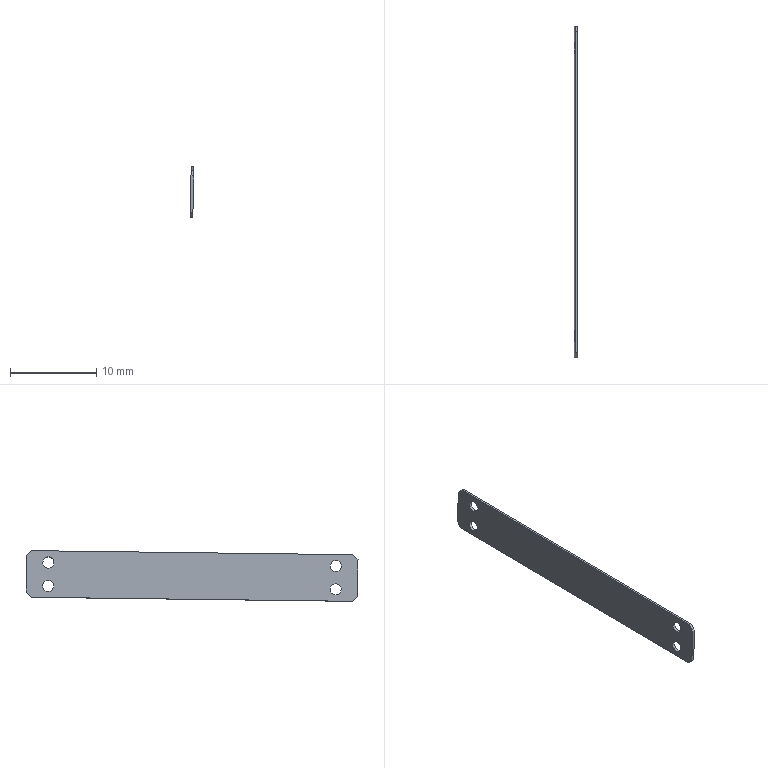Component | SolidWorks | 00-VacuumSuctionCupAssembly-1_11-RetainingPlate-2 | 1 solid | 18 faces | box 0.4 x 38.45 x 5.87 mm | volume 60 mm3 | plane 10 | cylinder 8 | commonest cylinder face diameters 1.29 x8
build123d program:
from build123d import *

# Parameters (mm, degrees)
SKETCH1_R           = 2.15
BOSS_EXTRUDE1_DEPTH = 1
SCALE1_SCALE        = 0.3


with BuildPart() as part:
    # Sketch1 → Boss-Extrude1 (new body)
    with BuildSketch(Plane(origin=(1, 0, 0), x_dir=(0, 0, -1), z_dir=(1, 0, 0))):
        Polygon((-64, 7), (-64, -7), (-62, -9), (62, -9), (64, -7), (64, 7), (62, 9), (-62, 9), align=None)
        with Locations(Location((-55.5, 4.5, 0), (0, 0, 180))):
            Circle(SKETCH1_R, mode=Mode.SUBTRACT)
        with Locations(Location((-55.5, -4.5, 0), (0, 0, 180))):
            Circle(SKETCH1_R, mode=Mode.SUBTRACT)
        with Locations(Location((55.5, 4.5, 0), (0, 0, 180))):
            Circle(SKETCH1_R, mode=Mode.SUBTRACT)
        with Locations(Location((55.5, -4.5, 0), (0, 0, 180))):
            Circle(SKETCH1_R, mode=Mode.SUBTRACT)
    extrude(amount=-BOSS_EXTRUDE1_DEPTH)


with BuildPart() as part_1:
    # Scale1: scaled about (0.5, 0, 0)
    add(part.part.scale(SCALE1_SCALE).moved(Location((0.35, 0, 0))))


solid = part_1.part

# Placed as in the assembly
solid = solid.moved(Location((72.646, 133.614, 48.988), (-89.279, 0.01259, -179)))